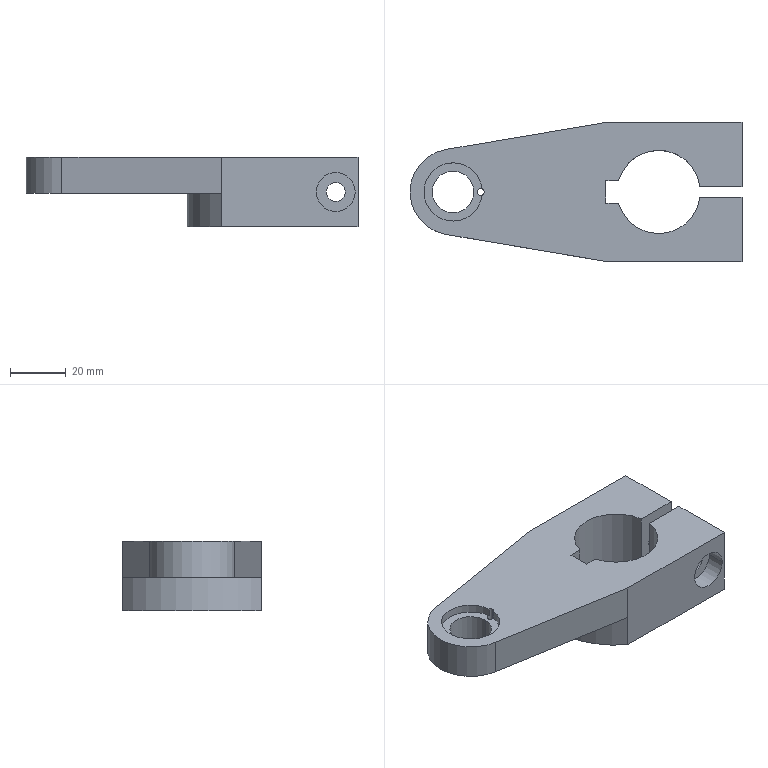CAM job | Mastercam | mm | 11 operations | part box 131.65 x 58.2 x 25
1. Facing | 6 - 10 平铣刀
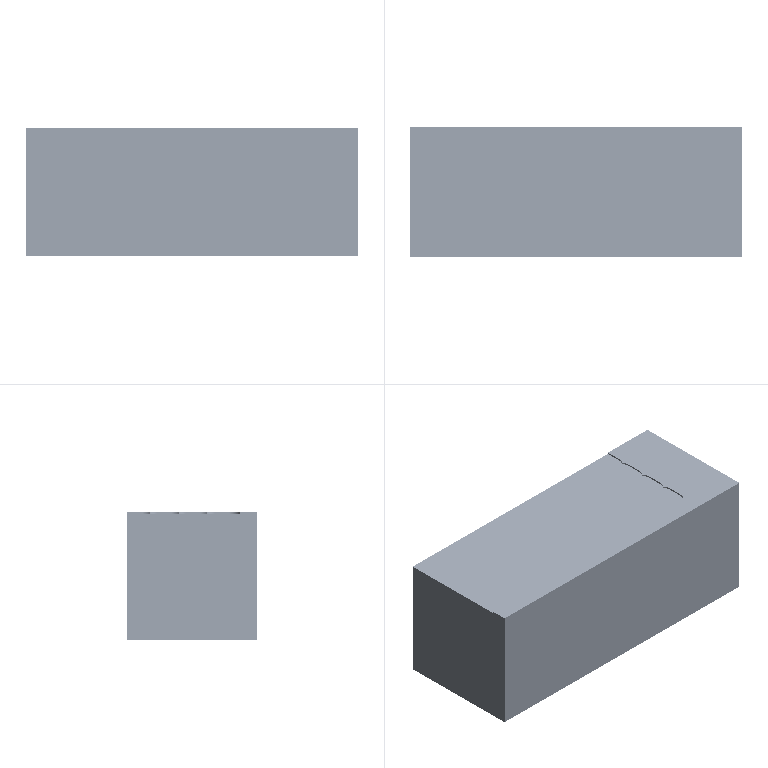2. Contour (Ramp) | 6 - 10 平铣刀
3. Contour (2D) | 6 - 10 平铣刀
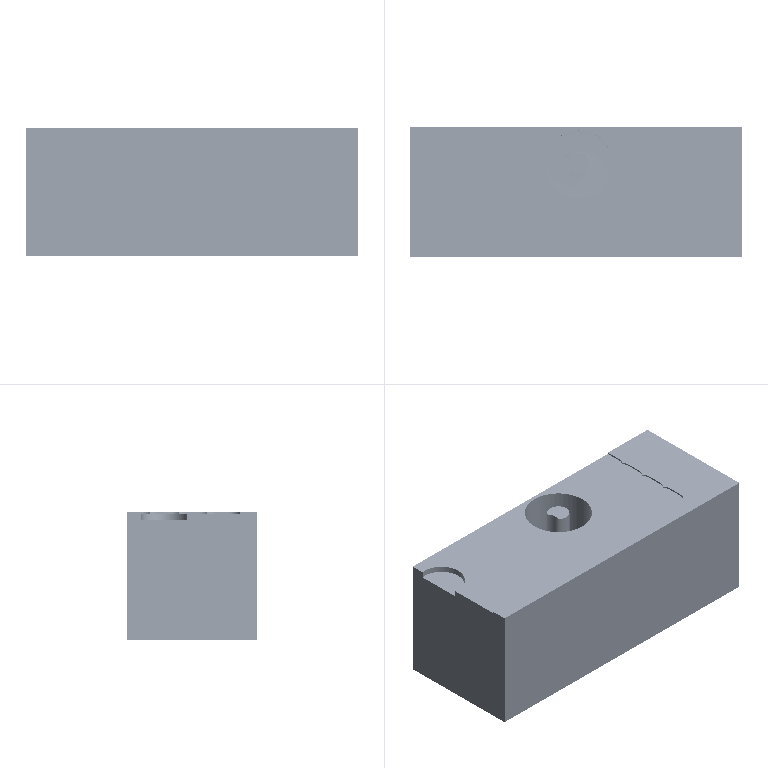4. Drill/Counterbore | 22 - 3 平铣刀
5. Peck Drill | 15 - 3 定位钻
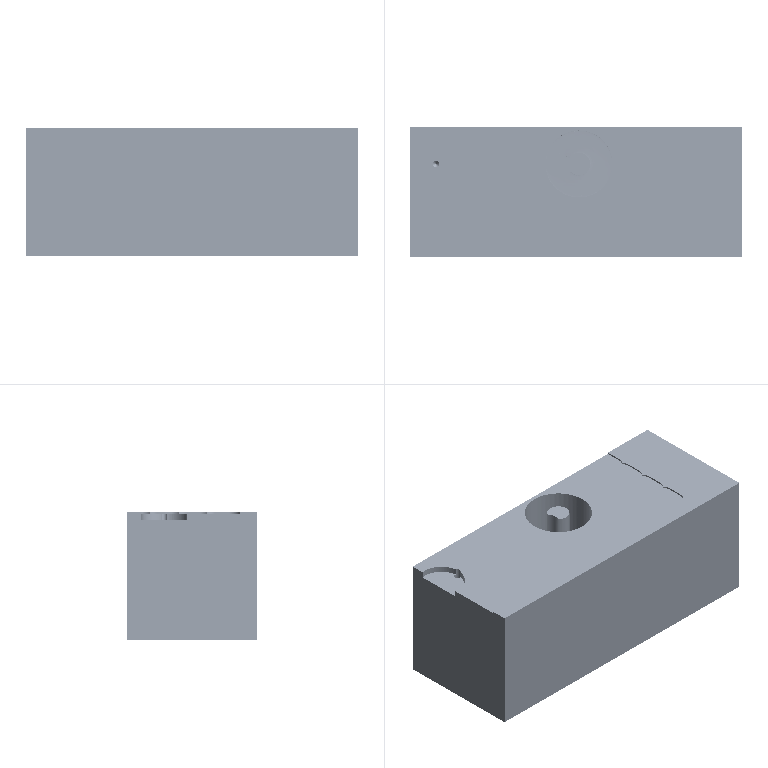6. Contour (2D) | 6 - 10 平铣刀
7. Contour (2D chamfer) | 2 - 6 倒角刀
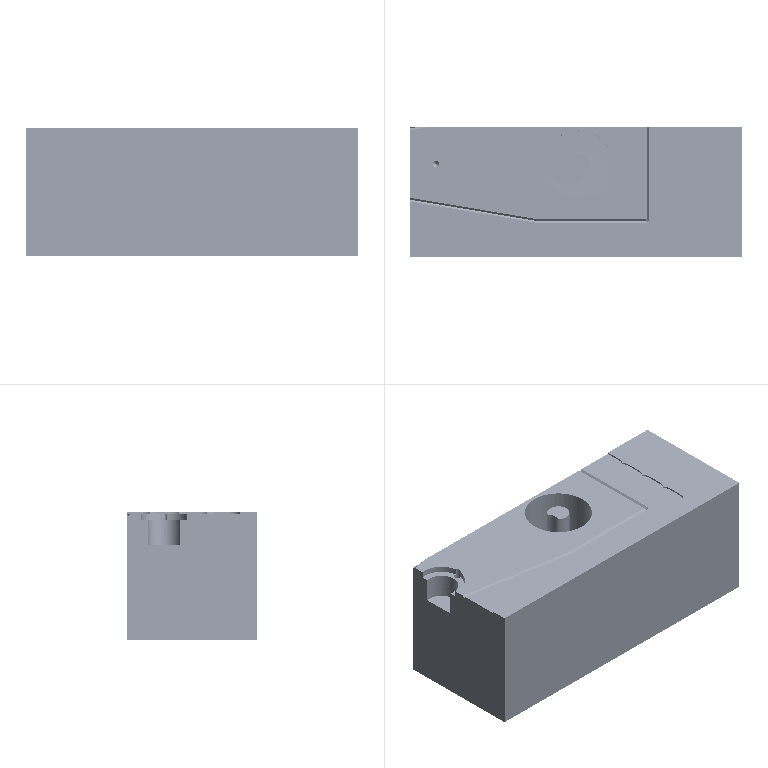8. Contour (2D chamfer) | 2 - 6 倒角刀
9. Drill/Counterbore | 2 - 6 倒角刀
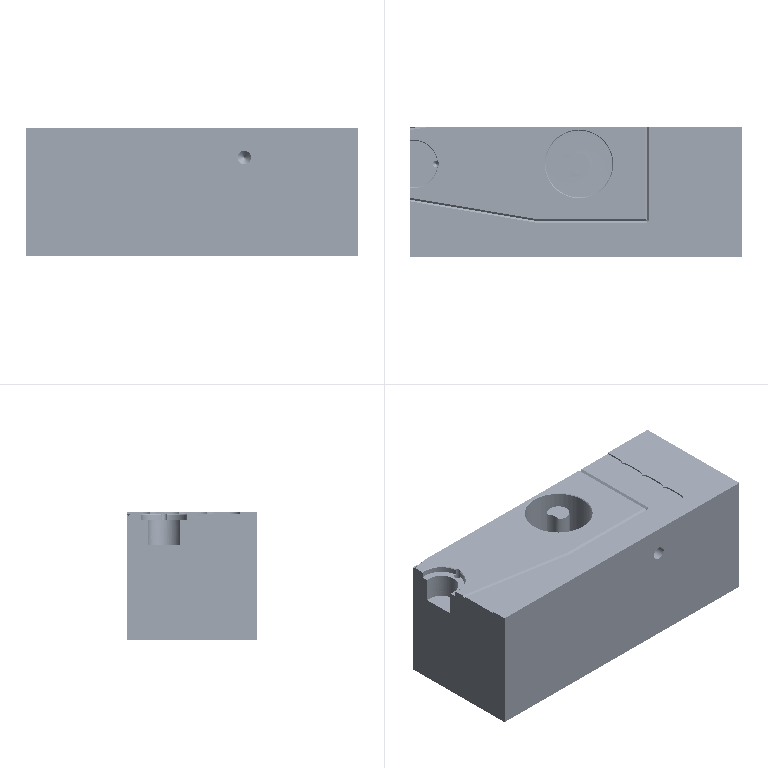10. Peck Drill | 1 - 6.8 钻头
11. 2D High Speed (2D Dynamic Mill) | 6 - 10 平铣刀